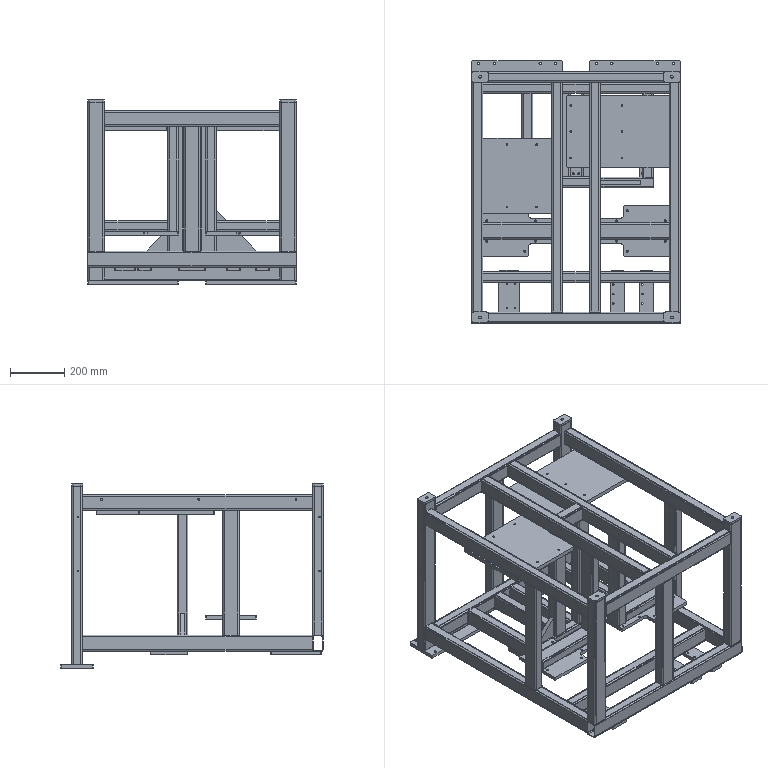Assembly | SolidWorks | mm | 19 component files | 50 solids | 946 faces | box 770 x 970 x 683 mm | volume 16294726 mm3 | plane 489 | cylinder 457 | commonest cylinder face diameters 12.8 x144 6.4 x128 6.8 x116 9 x32 6.6 x16 5 x8 10.2 x8 20 x4
Bill of materials:
STE21014.01-01 | 1 | Q235 | Open rectangular box-shaped frame built from square/rectangular-section straight bar members: four corner posts, top and bottom perimeter rails, intermediate vertical posts, and internal cross members including a smaller inset U-shaped sub-frame near the top.
STE21014.01-39 | 1 | Q235 | Thick rectangular plate with small chamfered corners and four through holes arranged as two pairs along the long axis.
STE21014.01-40 | 2 | Q235 | Elongated rectangular bar/plate with chamfered corners and four equally spaced through holes in a single row offset toward one long edge.
STE21014.01-41 | 2 | Q235 | Rectangular plate with chamfered corners and four equally spaced through holes in a single row offset toward one long edge; wider than the similar bar with four holes.
STE21014.01-42 | 2 | Q235 | Thin rectangular plate with small chamfered corners and eight through holes arranged as four pairs near the two long edges, grouped toward each end.
STE21014.01-43 | 1 | Q235 | Rectangular plate with chamfered corners and eight through holes arranged in a 2 x 4 grid along the centerline region.
STE21014.01-44 | 2 | Q235 | Thin plate with a stepped T-like/cross-shaped outline: a large square-ish main region with a narrower rectangular tongue extending from one side, with filleted inside corners, chamfered outer corners, and eight through holes.
STE21014.01-45 | 1 | Q235 | Thin, nearly rectangular plate with a rectangular notch removed from one corner (L-shaped outline), filleted inside corner, small chamfered corners, and four small through holes in a rectangular pattern.
STE21014.01-46 | 1 | Q235 | Flat right-triangle plate of uniform thickness with no visible holes; gusset-like shape.
STE21014.01-47 | 1 | Q235 | Flat right-triangle plate of uniform thickness with no visible holes; appears thicker relative to size than the other triangular plate and mirrored in orientation.
STE21014.01-48 | 1 | Q235 | Large thin rectangular plate with small chamfered corners and six small through holes arranged in a 2 x 3 pattern offset toward one end.
STE21014.03-29 | 4 | Q235 | Small thick rectangular block/plate with generously rounded vertical corners and a single central round through hole; washer-plate or spacer-like shape.
Mates:
1. coincident | STE21014.01-01-1 face at (0, 13.6, -610) dir (0, 0, -1) | STE21014.01-39-1 face at (107.5, 80, -610) dir (0, 0, 1)
2. distance | STE21014.01-01-1 face at (0, -20, -556.4) dir (0, -1, 0) | STE21014.01-39-1 face at (70, -15, -623) dir (0, -1, 0)
3. distance | STE21014.01-39-1 face at (70, 175, -623) dir (-1, 0, 0) | STE21014.01-01-1 face at (-30, 890, -556.4) dir (-1, 0, 0)
4. coincident | STE21014.01-01-1 face at (0, 13.6, -610) dir (0, 0, -1) | STE21014.01-40-1 face at (508.25, 80, -610) dir (0, 0, 1)
5. distance | STE21014.01-40-1 face at (482.25, -15, -623) dir (0, -1, 0) | STE21014.01-01-1 face at (0, -20, -556.4) dir (0, -1, 0)
6. distance | STE21014.01-40-1 face at (534.25, 175, -623) dir (1, 0, 0) | STE21014.01-01-1 face at (740, 890, -603.6) dir (1, 0, 0)
7. coincident | STE21014.01-01-1 face at (0, 13.6, -610) dir (0, 0, -1) | STE21014.01-40-2 face at (616.25, 80, -610) dir (0, 0, 1)
8. coincident | STE21014.01-40-1 face at (482.25, -15, -623) dir (0, -1, 0) | STE21014.01-40-2 face at (590.25, -15, -623) dir (0, -1, 0)
9. distance | STE21014.01-40-1 face at (534.25, 175, -623) dir (1, 0, 0) | STE21014.01-40-2 face at (642.25, 175, -623) dir (1, 0, 0)
10. coincident | STE21014.01-01-1 face at (633.6, 830, -610) dir (0, 0, -1) | STE21014.01-41-1 face at (615, 550, -610) dir (0, 0, 1)
11. coincident | STE21014.01-01-1 face at (175, 480, -556.4) dir (0, -1, 0) | STE21014.01-41-1 face at (590, 480, -610) dir (0, -1, 0)
12. coincident | STE21014.01-01-1 face at (188.6, 830, -610) dir (0, 0, -1) | STE21014.01-41-3 face at (180, 550, -610) dir (0, 0, 1)
13. coincident | STE21014.01-01-1 face at (0, 903.6, -660) dir (0, 0, -1) | STE21014.01-42-1 face at (572.5, 890, -660) dir (0, 0, 1)
14. distance | STE21014.01-01-1 face at (686.4, 910, 0) dir (0, 1, 0) | STE21014.01-42-1 face at (740, 950, -673) dir (0, 1, 0)
15. coincident | STE21014.01-01-1 face at (740, 876.4, 0) dir (1, 0, 0) | STE21014.01-42-1 face at (740, 950, -673) dir (1, 0, 0)
16. coincident | STE21014.01-42-1 face at (572.5, 890, -673) dir (0, 0, -1) | STE21014.01-42-2 face at (137.5, 890, -673) dir (0, 0, -1)
17. coincident | STE21014.01-42-1 face at (740, 830, -673) dir (0, -1, 0) | STE21014.01-42-2 face at (305, 830, -673) dir (0, -1, 0)
18. coincident | STE21014.01-01-1 face at (-30, 903.6, 0) dir (-1, 0, 0) | STE21014.01-42-2 face at (-30, 950, -673) dir (-1, 0, 0)
19. coincident | STE21014.01-01-1 face at (405, 296.9, -60) dir (-1, 0, 0) | STE21014.01-44-1 face at (405, 226.5, -478) dir (-1, 0, 0)
20. coincident | STE21014.01-01-1 face at (710, 344.1, -478) dir (0, 0, -1) | STE21014.01-44-1 face at (552.5, 320.5, -478) dir (0, 0, 1)
21. distance | STE21014.01-01-1 face at (710, 290.5, -444.4) dir (0, -1, 0) | STE21014.01-44-1 face at (700, 226.5, -478) dir (0, -1, 0)
22. coincident | STE21014.01-01-1 face at (285, 344.1, -478) dir (0, 0, -1) | STE21014.01-44-2 face at (157.5, 320.5, -478) dir (0, 0, 1)
23. coincident | STE21014.01-01-1 face at (305, 344.1, -60) dir (1, 0, 0) | STE21014.01-44-2 face at (305, 414.5, -478) dir (1, 0, 0)
24. coincident | STE21014.01-44-1 face at (700, 226.5, -478) dir (0, -1, 0) | STE21014.01-44-2 face at (10, 226.5, -478) dir (0, -1, 0)
25. coincident | STE21014.01-01-1 face at (3.6, 890, -90) dir (0, 0, -1) | STE21014.01-45-1 face at (137.5, 523.5, -90) dir (0, 0, 1)
26. distance | STE21014.01-45-1 face at (305, 383.5, -105) dir (0, -1, 0) | STE21014.01-01-1 face at (0, -20, -36.4) dir (0, -1, 0)
27. coincident | STE21014.01-01-1 face at (-30, 890, -36.4) dir (-1, 0, 0) | STE21014.01-45-1 face at (-30, 663.5, -105) dir (-1, 0, 0)
28. coincident | STE21014.01-01-1 face at (445, 486.4, -60) dir (1, 0, 0) | STE21014.01-46-1 face at (445, 507.5, -550) dir (-1, 0, 0)
29. coincident | STE21014.01-01-1 face at (175, 486.4, -550) dir (0, 0, 1) | STE21014.01-46-1 face at (445, 507.5, -550) dir (0, 0, -1)
30. width | STE21014.01-01-1 face at (391.4, 520, -60) dir (0, 1, 0) | STE21014.01-01-1 face at (438.6, 480, -60) dir (0, -1, 0) | STE21014.01-46-1 face at (445, 492.5, -550) dir (0, -1, 0) | STE21014.01-46-1 face at (445, 507.5, -550) dir (0, 1, 0)
31. coincident | STE21014.01-01-1 face at (265, 513.6, -60) dir (-1, 0, 0) | STE21014.01-47-1 face at (265, 492.5, -550) dir (1, 0, 0)
32. coincident | STE21014.01-01-1 face at (175, 486.4, -550) dir (0, 0, 1) | STE21014.01-47-1 face at (265, 492.5, -550) dir (0, 0, -1)
33. width | STE21014.01-01-1 face at (271.4, 520, -60) dir (0, 1, 0) | STE21014.01-01-1 face at (318.6, 480, -60) dir (0, -1, 0) | STE21014.01-47-1 face at (265, 492.5, -550) dir (0, -1, 0) | STE21014.01-47-1 face at (265, 507.5, -550) dir (0, 1, 0)
34. coincident | STE21014.01-01-1 face at (733.6, 890, -90) dir (0, 0, -1) | STE21014.01-48-1 face at (530, 687.5, -90) dir (0, 0, 1)
35. coincident | STE21014.01-01-1 face at (740, 890, -83.6) dir (1, 0, 0) | STE21014.01-48-1 face at (740, 820, -90) dir (1, 0, 0)
36. distance | STE21014.01-48-1 face at (320, 820, -90) dir (0, 1, 0) | STE21014.01-01-1 face at (0, 910, -83.6) dir (0, 1, 0)
37. coincident | STE21014.01-01-1 face at (640, 500, -550) dir (1, 0, 0) | STE21014.01-41-1 face at (640, 480, -610) dir (1, 0, 0)
38. coincident | STE21014.01-01-1 face at (155, 500, -610) dir (-1, 0, 0) | STE21014.01-41-3 face at (155, 480, -610) dir (-1, 0, 0)
39. coincident | STE21014.01-01-1 face at (408.6, 830, -610) dir (0, 0, -1) | STE21014.01-43-1 face at (355, 550, -610) dir (0, 0, 1)
40. coincident | STE21014.01-01-1 face at (175, 480, -556.4) dir (0, -1, 0) | STE21014.01-43-1 face at (305, 480, -623) dir (0, -1, 0)
41. distance | STE21014.01-43-1 face at (405, 620, -623) dir (1, 0, 0) | STE21014.01-01-1 face at (415, 830, -603.6) dir (1, 0, 0)
42. distance | STE21014.01-41-3 face at (155, 480, -610) dir (0, -1, 0) | STE21014.01-01-1 face at (175, 480, -556.4) dir (0, -1, 0)
43. coincident | STE21014.01-01-1 face at (-23.6, 13.6, 0) dir (0, 0, 1) | STE21014.03-29-1 face at (0, 0, 0) dir (0, 0, -1)
44. coincident | STE21014.01-01-1 face at (23.6, -20, 0) dir (0, -1, 0) | STE21014.03-29-1 face at (30, -20, 0) dir (0, -1, 0)
45. coincident | STE21014.01-01-1 face at (-30, 13.6, 0) dir (-1, 0, 0) | STE21014.03-29-1 face at (-30, -20, 0) dir (-1, 0, 0)
46. coincident | STE21014.01-01-1 face at (686.4, 13.6, 0) dir (0, 0, 1) | STE21014.03-29-2 face at (710, 0, 0) dir (0, 0, -1)
47. coincident | STE21014.01-01-1 face at (733.6, -20, 0) dir (0, -1, 0) | STE21014.03-29-2 face at (740, -20, 0) dir (0, -1, 0)
48. coincident | STE21014.01-01-1 face at (680, 13.6, 0) dir (-1, 0, 0) | STE21014.03-29-2 face at (680, -20, 0) dir (-1, 0, 0)
49. coincident | STE21014.01-01-1 face at (-23.6, 903.6, 0) dir (0, 0, 1) | STE21014.03-29-3 face at (0, 890, 0) dir (0, 0, -1)
50. coincident | STE21014.01-01-1 face at (23.6, 870, 0) dir (0, -1, 0) | STE21014.03-29-3 face at (30, 870, 0) dir (0, -1, 0)
51. coincident | STE21014.01-01-1 face at (-30, 903.6, 0) dir (-1, 0, 0) | STE21014.03-29-3 face at (-30, 870, 0) dir (-1, 0, 0)
52. coincident | STE21014.01-01-1 face at (686.4, 903.6, 0) dir (0, 0, 1) | STE21014.03-29-4 face at (710, 890, 0) dir (0, 0, -1)
53. coincident | STE21014.01-01-1 face at (733.6, 870, 0) dir (0, -1, 0) | STE21014.03-29-4 face at (740, 870, 0) dir (0, -1, 0)
54. coincident | STE21014.01-01-1 face at (680, 903.6, 0) dir (-1, 0, 0) | STE21014.03-29-4 face at (680, 870, 0) dir (-1, 0, 0)